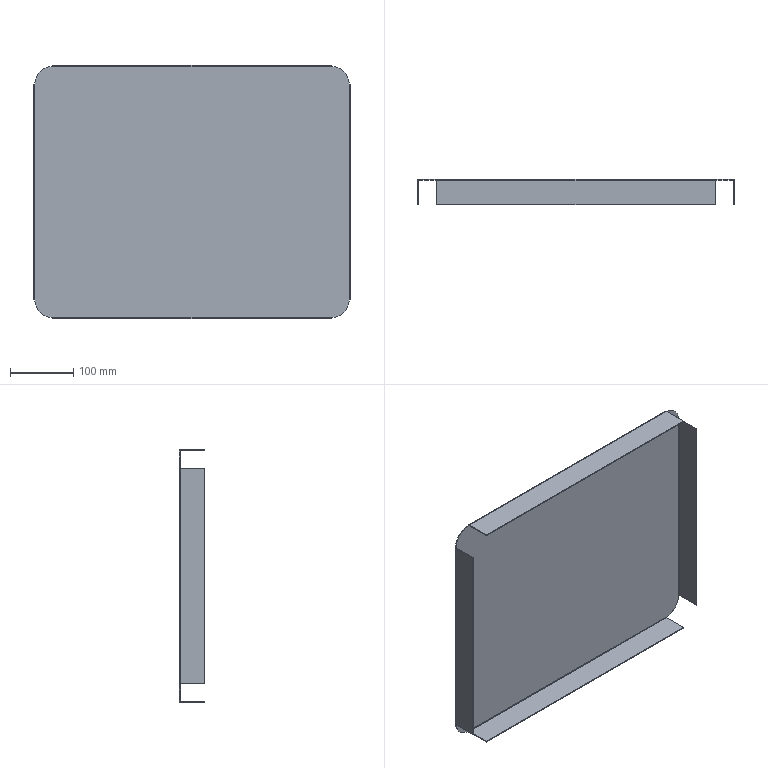Component | SolidWorks | dbj3-1_w11-1 | 1 solid | 42 faces | box 500 x 40 x 400 mm | volume 387129 mm3 | plane 30 | cylinder 12 | commonest cylinder face diameters 56 x4 4 x4 1 x4
STEP:
#1=COLOUR_RGB('',0.7922,0.8196,0.9333);
#2=FILL_AREA_STYLE_COLOUR('',#1);
#3=FILL_AREA_STYLE('',(#2));
#4=SURFACE_STYLE_FILL_AREA(#3);
#5=SURFACE_SIDE_STYLE('',(#4));
#6=SURFACE_STYLE_USAGE(.BOTH.,#5);
#7=PRESENTATION_STYLE_ASSIGNMENT((#6));
#8=CARTESIAN_POINT('',(-9.764,-29.498,8.661));
#9=VERTEX_POINT('',#8);
#10=CARTESIAN_POINT('',(-8.661,-29.498,9.764));
#11=VERTEX_POINT('',#10);
#12=CARTESIAN_POINT('',(-8.661,-29.498,8.661));
#13=DIRECTION('',(0.,1.,-0.));
#14=DIRECTION('',(1.,0.,0.));
#15=AXIS2_PLACEMENT_3D('',#12,#13,#14);
#16=CIRCLE('',#15,1.102);
#17=EDGE_CURVE('',#9,#11,#16,.T.);
#18=ORIENTED_EDGE('',*,*,#17,.F.);
#19=CARTESIAN_POINT('',(-9.764,-29.557,8.661));
#20=VERTEX_POINT('',#19);
#21=CARTESIAN_POINT('',(-9.764,-29.557,8.661));
#22=DIRECTION('',(0.,1.,-0.));
#23=VECTOR('',#22,39.37);
#24=LINE('',#21,#23);
#25=EDGE_CURVE('',#20,#9,#24,.T.);
#26=ORIENTED_EDGE('',*,*,#25,.F.);
#27=CARTESIAN_POINT('',(-8.661,-29.557,9.764));
#28=VERTEX_POINT('',#27);
#29=CARTESIAN_POINT('',(-8.661,-29.557,8.661));
#30=DIRECTION('',(0.,1.,-0.));
#31=DIRECTION('',(1.,0.,0.));
#32=AXIS2_PLACEMENT_3D('',#29,#30,#31);
#33=CIRCLE('',#32,1.102);
#34=EDGE_CURVE('',#20,#28,#33,.T.);
#35=ORIENTED_EDGE('',*,*,#34,.T.);
#36=CARTESIAN_POINT('',(-8.661,-29.557,9.764));
#37=DIRECTION('',(0.,1.,-0.));
#38=VECTOR('',#37,39.37);
#39=LINE('',#36,#38);
#40=EDGE_CURVE('',#28,#11,#39,.T.);
#41=ORIENTED_EDGE('',*,*,#40,.T.);
#42=EDGE_LOOP('',(#18,#26,#35,#41));
#43=FACE_OUTER_BOUND('',#42,.T.);
#44=CARTESIAN_POINT('',(-8.661,-29.557,8.661));
#45=DIRECTION('',(0.,1.,-0.));
#46=DIRECTION('',(1.,0.,0.));
#47=AXIS2_PLACEMENT_3D('',#44,#45,#46);
#48=CYLINDRICAL_SURFACE('',#47,1.102);
#49=ADVANCED_FACE('',(#43),#48,.T.);
#50=CARTESIAN_POINT('',(-8.661,-29.498,-5.827));
#51=VERTEX_POINT('',#50);
#52=CARTESIAN_POINT('',(-9.764,-29.498,-4.724));
#53=VERTEX_POINT('',#52);
#54=CARTESIAN_POINT('',(-8.661,-29.498,-4.724));
#55=DIRECTION('',(0.,1.,-0.));
#56=DIRECTION('',(1.,0.,0.));
#57=AXIS2_PLACEMENT_3D('',#54,#55,#56);
#58=CIRCLE('',#57,1.102);
#59=EDGE_CURVE('',#51,#53,#58,.T.);
#60=ORIENTED_EDGE('',*,*,#59,.F.);
#61=CARTESIAN_POINT('',(-8.661,-29.557,-5.827));
#62=VERTEX_POINT('',#61);
#63=CARTESIAN_POINT('',(-8.661,-29.557,-5.827));
#64=DIRECTION('',(0.,1.,-0.));
#65=VECTOR('',#64,39.37);
#66=LINE('',#63,#65);
#67=EDGE_CURVE('',#62,#51,#66,.T.);
#68=ORIENTED_EDGE('',*,*,#67,.F.);
#69=CARTESIAN_POINT('',(-9.764,-29.557,-4.724));
#70=VERTEX_POINT('',#69);
#71=CARTESIAN_POINT('',(-8.661,-29.557,-4.724));
#72=DIRECTION('',(0.,1.,-0.));
#73=DIRECTION('',(1.,0.,0.));
#74=AXIS2_PLACEMENT_3D('',#71,#72,#73);
#75=CIRCLE('',#74,1.102);
#76=EDGE_CURVE('',#62,#70,#75,.T.);
#77=ORIENTED_EDGE('',*,*,#76,.T.);
#78=CARTESIAN_POINT('',(-9.764,-29.557,-4.724));
#79=DIRECTION('',(0.,1.,-0.));
#80=VECTOR('',#79,39.37);
#81=LINE('',#78,#80);
#82=EDGE_CURVE('',#70,#53,#81,.T.);
#83=ORIENTED_EDGE('',*,*,#82,.T.);
#84=EDGE_LOOP('',(#60,#68,#77,#83));
#85=FACE_OUTER_BOUND('',#84,.T.);
#86=CARTESIAN_POINT('',(-8.661,-29.557,-4.724));
#87=DIRECTION('',(0.,1.,-0.));
#88=DIRECTION('',(1.,0.,0.));
#89=AXIS2_PLACEMENT_3D('',#86,#87,#88);
#90=CYLINDRICAL_SURFACE('',#89,1.102);
#91=ADVANCED_FACE('',(#85),#90,.T.);
#92=CARTESIAN_POINT('',(9.764,-29.498,-4.724));
#93=VERTEX_POINT('',#92);
#94=CARTESIAN_POINT('',(8.661,-29.498,-5.827));
#95=VERTEX_POINT('',#94);
#96=CARTESIAN_POINT('',(8.661,-29.498,-4.724));
#97=DIRECTION('',(0.,1.,-0.));
#98=DIRECTION('',(1.,0.,0.));
#99=AXIS2_PLACEMENT_3D('',#96,#97,#98);
#100=CIRCLE('',#99,1.102);
#101=EDGE_CURVE('',#93,#95,#100,.T.);
#102=ORIENTED_EDGE('',*,*,#101,.F.);
#103=CARTESIAN_POINT('',(9.764,-29.557,-4.724));
#104=VERTEX_POINT('',#103);
#105=CARTESIAN_POINT('',(9.764,-29.557,-4.724));
#106=DIRECTION('',(0.,1.,-0.));
#107=VECTOR('',#106,39.37);
#108=LINE('',#105,#107);
#109=EDGE_CURVE('',#104,#93,#108,.T.);
#110=ORIENTED_EDGE('',*,*,#109,.F.);
#111=CARTESIAN_POINT('',(8.661,-29.557,-5.827));
#112=VERTEX_POINT('',#111);
#113=CARTESIAN_POINT('',(8.661,-29.557,-4.724));
#114=DIRECTION('',(0.,1.,-0.));
#115=DIRECTION('',(1.,0.,0.));
#116=AXIS2_PLACEMENT_3D('',#113,#114,#115);
#117=CIRCLE('',#116,1.102);
#118=EDGE_CURVE('',#104,#112,#117,.T.);
#119=ORIENTED_EDGE('',*,*,#118,.T.);
#120=CARTESIAN_POINT('',(8.661,-29.557,-5.827));
#121=DIRECTION('',(0.,1.,-0.));
#122=VECTOR('',#121,39.37);
#123=LINE('',#120,#122);
#124=EDGE_CURVE('',#112,#95,#123,.T.);
#125=ORIENTED_EDGE('',*,*,#124,.T.);
#126=EDGE_LOOP('',(#102,#110,#119,#125));
#127=FACE_OUTER_BOUND('',#126,.T.);
#128=CARTESIAN_POINT('',(8.661,-29.557,-4.724));
#129=DIRECTION('',(0.,1.,-0.));
#130=DIRECTION('',(1.,0.,0.));
#131=AXIS2_PLACEMENT_3D('',#128,#129,#130);
#132=CYLINDRICAL_SURFACE('',#131,1.102);
#133=ADVANCED_FACE('',(#127),#132,.T.);
#134=CARTESIAN_POINT('',(8.661,-29.498,9.764));
#135=VERTEX_POINT('',#134);
#136=CARTESIAN_POINT('',(9.764,-29.498,8.661));
#137=VERTEX_POINT('',#136);
#138=CARTESIAN_POINT('',(8.661,-29.498,8.661));
#139=DIRECTION('',(0.,1.,-0.));
#140=DIRECTION('',(1.,0.,0.));
#141=AXIS2_PLACEMENT_3D('',#138,#139,#140);
#142=CIRCLE('',#141,1.102);
#143=EDGE_CURVE('',#135,#137,#142,.T.);
#144=ORIENTED_EDGE('',*,*,#143,.F.);
#145=CARTESIAN_POINT('',(8.661,-29.557,9.764));
#146=VERTEX_POINT('',#145);
#147=CARTESIAN_POINT('',(8.661,-29.557,9.764));
#148=DIRECTION('',(0.,1.,-0.));
#149=VECTOR('',#148,39.37);
#150=LINE('',#147,#149);
#151=EDGE_CURVE('',#146,#135,#150,.T.);
#152=ORIENTED_EDGE('',*,*,#151,.F.);
#153=CARTESIAN_POINT('',(9.764,-29.557,8.661));
#154=VERTEX_POINT('',#153);
#155=CARTESIAN_POINT('',(8.661,-29.557,8.661));
#156=DIRECTION('',(0.,1.,-0.));
#157=DIRECTION('',(1.,0.,0.));
#158=AXIS2_PLACEMENT_3D('',#155,#156,#157);
#159=CIRCLE('',#158,1.102);
#160=EDGE_CURVE('',#146,#154,#159,.T.);
#161=ORIENTED_EDGE('',*,*,#160,.T.);
#162=CARTESIAN_POINT('',(9.764,-29.557,8.661));
#163=DIRECTION('',(0.,1.,-0.));
#164=VECTOR('',#163,39.37);
#165=LINE('',#162,#164);
#166=EDGE_CURVE('',#154,#137,#165,.T.);
#167=ORIENTED_EDGE('',*,*,#166,.T.);
#168=EDGE_LOOP('',(#144,#152,#161,#167));
#169=FACE_OUTER_BOUND('',#168,.T.);
#170=CARTESIAN_POINT('',(8.661,-29.557,8.661));
#171=DIRECTION('',(0.,1.,-0.));
#172=DIRECTION('',(1.,0.,0.));
#173=AXIS2_PLACEMENT_3D('',#170,#171,#172);
#174=CYLINDRICAL_SURFACE('',#173,1.102);
#175=ADVANCED_FACE('',(#169),#174,.T.);
#176=ORIENTED_EDGE('',*,*,#34,.F.);
#177=CARTESIAN_POINT('',(-9.764,-29.557,8.661));
#178=DIRECTION('',(0.,0.,1.));
#179=VECTOR('',#178,39.37);
#180=LINE('',#177,#179);
#181=EDGE_CURVE('',#70,#20,#180,.T.);
#182=ORIENTED_EDGE('',*,*,#181,.F.);
#183=ORIENTED_EDGE('',*,*,#76,.F.);
#184=CARTESIAN_POINT('',(8.661,-29.557,-5.827));
#185=DIRECTION('',(-1.,0.,0.));
#186=VECTOR('',#185,39.37);
#187=LINE('',#184,#186);
#188=EDGE_CURVE('',#112,#62,#187,.T.);
#189=ORIENTED_EDGE('',*,*,#188,.F.);
#190=ORIENTED_EDGE('',*,*,#118,.F.);
#191=CARTESIAN_POINT('',(9.764,-29.557,8.661));
#192=DIRECTION('',(-0.,-0.,-1.));
#193=VECTOR('',#192,39.37);
#194=LINE('',#191,#193);
#195=EDGE_CURVE('',#154,#104,#194,.T.);
#196=ORIENTED_EDGE('',*,*,#195,.F.);
#197=ORIENTED_EDGE('',*,*,#160,.F.);
#198=CARTESIAN_POINT('',(8.661,-29.557,9.764));
#199=DIRECTION('',(1.,-0.,-0.));
#200=VECTOR('',#199,39.37);
#201=LINE('',#198,#200);
#202=EDGE_CURVE('',#28,#146,#201,.T.);
#203=ORIENTED_EDGE('',*,*,#202,.F.);
#204=EDGE_LOOP('',(#176,#182,#183,#189,#190,#196,#197,#203));
#205=FACE_OUTER_BOUND('',#204,.T.);
#206=CARTESIAN_POINT('',(-8.661,-29.557,8.661));
#207=DIRECTION('',(0.,1.,-0.));
#208=DIRECTION('',(1.,-0.,-0.));
#209=AXIS2_PLACEMENT_3D('',#206,#207,#208);
#210=PLANE('',#209);
#211=ADVANCED_FACE('',(#205),#210,.F.);
#212=ORIENTED_EDGE('',*,*,#17,.T.);
#213=CARTESIAN_POINT('',(8.661,-29.498,9.764));
#214=DIRECTION('',(1.,-0.,-0.));
#215=VECTOR('',#214,39.37);
#216=LINE('',#213,#215);
#217=EDGE_CURVE('',#11,#135,#216,.T.);
#218=ORIENTED_EDGE('',*,*,#217,.T.);
#219=ORIENTED_EDGE('',*,*,#143,.T.);
#220=CARTESIAN_POINT('',(9.764,-29.498,8.661));
#221=DIRECTION('',(-0.,-0.,-1.));
#222=VECTOR('',#221,39.37);
#223=LINE('',#220,#222);
#224=EDGE_CURVE('',#137,#93,#223,.T.);
#225=ORIENTED_EDGE('',*,*,#224,.T.);
#226=ORIENTED_EDGE('',*,*,#101,.T.);
#227=CARTESIAN_POINT('',(8.661,-29.498,-5.827));
#228=DIRECTION('',(-1.,0.,0.));
#229=VECTOR('',#228,39.37);
#230=LINE('',#227,#229);
#231=EDGE_CURVE('',#95,#51,#230,.T.);
#232=ORIENTED_EDGE('',*,*,#231,.T.);
#233=ORIENTED_EDGE('',*,*,#59,.T.);
#234=CARTESIAN_POINT('',(-9.764,-29.498,8.661));
#235=DIRECTION('',(0.,0.,1.));
#236=VECTOR('',#235,39.37);
#237=LINE('',#234,#236);
#238=EDGE_CURVE('',#53,#9,#237,.T.);
#239=ORIENTED_EDGE('',*,*,#238,.T.);
#240=EDGE_LOOP('',(#212,#218,#219,#225,#226,#232,#233,#239));
#241=FACE_OUTER_BOUND('',#240,.T.);
#242=CARTESIAN_POINT('',(-8.661,-29.498,8.661));
#243=DIRECTION('',(0.,1.,-0.));
#244=DIRECTION('',(1.,-0.,-0.));
#245=AXIS2_PLACEMENT_3D('',#242,#243,#244);
#246=PLANE('',#245);
#247=ADVANCED_FACE('',(#241),#246,.T.);
#248=CARTESIAN_POINT('',(-8.661,-29.577,-5.846));
#249=VERTEX_POINT('',#248);
#250=CARTESIAN_POINT('',(-8.661,-29.577,-5.906));
#251=VERTEX_POINT('',#250);
#252=CARTESIAN_POINT('',(-8.661,-29.577,-5.906));
#253=DIRECTION('',(-0.,0.,-1.));
#254=VECTOR('',#253,39.37);
#255=LINE('',#252,#254);
#256=EDGE_CURVE('',#249,#251,#255,.T.);
#257=ORIENTED_EDGE('',*,*,#256,.F.);
#258=CARTESIAN_POINT('',(-8.661,-29.577,-5.827));
#259=DIRECTION('',(-1.,0.,0.));
#260=DIRECTION('',(0.,-1.,0.));
#261=AXIS2_PLACEMENT_3D('',#258,#259,#260);
#262=CIRCLE('',#261,0.01969);
#263=EDGE_CURVE('',#62,#249,#262,.T.);
#264=ORIENTED_EDGE('',*,*,#263,.F.);
#265=ORIENTED_EDGE('',*,*,#67,.T.);
#266=CARTESIAN_POINT('',(-8.661,-29.577,-5.827));
#267=DIRECTION('',(-1.,0.,0.));
#268=DIRECTION('',(0.,-1.,0.));
#269=AXIS2_PLACEMENT_3D('',#266,#267,#268);
#270=CIRCLE('',#269,0.07874);
#271=EDGE_CURVE('',#51,#251,#270,.T.);
#272=ORIENTED_EDGE('',*,*,#271,.T.);
#273=EDGE_LOOP('',(#257,#264,#265,#272));
#274=FACE_OUTER_BOUND('',#273,.T.);
#275=CARTESIAN_POINT('',(-8.661,-29.577,-5.827));
#276=DIRECTION('',(-1.,0.,0.));
#277=DIRECTION('',(0.,1.,-0.));
#278=AXIS2_PLACEMENT_3D('',#275,#276,#277);
#279=PLANE('',#278);
#280=ADVANCED_FACE('',(#274),#279,.T.);
#281=CARTESIAN_POINT('',(8.661,-29.577,-5.846));
#282=VERTEX_POINT('',#281);
#283=CARTESIAN_POINT('',(8.661,-29.577,-5.827));
#284=DIRECTION('',(1.,-0.,-0.));
#285=DIRECTION('',(0.,-1.,0.));
#286=AXIS2_PLACEMENT_3D('',#283,#284,#285);
#287=CIRCLE('',#286,0.01969);
#288=EDGE_CURVE('',#282,#112,#287,.T.);
#289=ORIENTED_EDGE('',*,*,#288,.F.);
#290=CARTESIAN_POINT('',(8.661,-29.577,-5.906));
#291=VERTEX_POINT('',#290);
#292=CARTESIAN_POINT('',(8.661,-29.577,-5.846));
#293=DIRECTION('',(-0.,0.,-1.));
#294=VECTOR('',#293,39.37);
#295=LINE('',#292,#294);
#296=EDGE_CURVE('',#282,#291,#295,.T.);
#297=ORIENTED_EDGE('',*,*,#296,.T.);
#298=CARTESIAN_POINT('',(8.661,-29.577,-5.827));
#299=DIRECTION('',(1.,-0.,-0.));
#300=DIRECTION('',(0.,-1.,0.));
#301=AXIS2_PLACEMENT_3D('',#298,#299,#300);
#302=CIRCLE('',#301,0.07874);
#303=EDGE_CURVE('',#291,#95,#302,.T.);
#304=ORIENTED_EDGE('',*,*,#303,.T.);
#305=ORIENTED_EDGE('',*,*,#124,.F.);
#306=EDGE_LOOP('',(#289,#297,#304,#305));
#307=FACE_OUTER_BOUND('',#306,.T.);
#308=CARTESIAN_POINT('',(8.661,-29.577,-5.827));
#309=DIRECTION('',(-1.,0.,0.));
#310=DIRECTION('',(0.,1.,-0.));
#311=AXIS2_PLACEMENT_3D('',#308,#309,#310);
#312=PLANE('',#311);
#313=ADVANCED_FACE('',(#307),#312,.F.);
#314=ORIENTED_EDGE('',*,*,#231,.F.);
#315=ORIENTED_EDGE('',*,*,#303,.F.);
#316=CARTESIAN_POINT('',(-8.661,-29.577,-5.906));
#317=DIRECTION('',(-1.,0.,0.));
#318=VECTOR('',#317,39.37);
#319=LINE('',#316,#318);
#320=EDGE_CURVE('',#291,#251,#319,.T.);
#321=ORIENTED_EDGE('',*,*,#320,.T.);
#322=ORIENTED_EDGE('',*,*,#271,.F.);
#323=EDGE_LOOP('',(#314,#315,#321,#322));
#324=FACE_OUTER_BOUND('',#323,.T.);
#325=CARTESIAN_POINT('',(8.661,-29.577,-5.827));
#326=DIRECTION('',(1.,-0.,-0.));
#327=DIRECTION('',(0.,0.,-1.));
#328=AXIS2_PLACEMENT_3D('',#325,#326,#327);
#329=CYLINDRICAL_SURFACE('',#328,0.07874);
#330=ADVANCED_FACE('',(#324),#329,.T.);
#331=ORIENTED_EDGE('',*,*,#188,.T.);
#332=ORIENTED_EDGE('',*,*,#263,.T.);
#333=CARTESIAN_POINT('',(-8.661,-29.577,-5.846));
#334=DIRECTION('',(1.,-0.,-0.));
#335=VECTOR('',#334,39.37);
#336=LINE('',#333,#335);
#337=EDGE_CURVE('',#249,#282,#336,.T.);
#338=ORIENTED_EDGE('',*,*,#337,.T.);
#339=ORIENTED_EDGE('',*,*,#288,.T.);
#340=EDGE_LOOP('',(#331,#332,#338,#339));
#341=FACE_OUTER_BOUND('',#340,.T.);
#342=CARTESIAN_POINT('',(8.661,-29.577,-5.827));
#343=DIRECTION('',(1.,-0.,-0.));
#344=DIRECTION('',(0.,0.,-1.));
#345=AXIS2_PLACEMENT_3D('',#342,#343,#344);
#346=CYLINDRICAL_SURFACE('',#345,0.01969);
#347=ADVANCED_FACE('',(#341),#346,.F.);
#348=ORIENTED_EDGE('',*,*,#296,.F.);
#349=CARTESIAN_POINT('',(8.661,-31.073,-5.846));
#350=VERTEX_POINT('',#349);
#351=CARTESIAN_POINT('',(8.661,-31.073,-5.846));
#352=DIRECTION('',(-0.,-1.,-0.));
#353=VECTOR('',#352,39.37);
#354=LINE('',#351,#353);
#355=EDGE_CURVE('',#282,#350,#354,.T.);
#356=ORIENTED_EDGE('',*,*,#355,.T.);
#357=CARTESIAN_POINT('',(8.661,-31.073,-5.906));
#358=VERTEX_POINT('',#357);
#359=CARTESIAN_POINT('',(8.661,-31.073,-5.906));
#360=DIRECTION('',(0.,0.,1.));
#361=VECTOR('',#360,39.37);
#362=LINE('',#359,#361);
#363=EDGE_CURVE('',#358,#350,#362,.T.);
#364=ORIENTED_EDGE('',*,*,#363,.F.);
#365=CARTESIAN_POINT('',(8.661,-29.498,-5.906));
#366=DIRECTION('',(-0.,-1.,-0.));
#367=VECTOR('',#366,39.37);
#368=LINE('',#365,#367);
#369=EDGE_CURVE('',#291,#358,#368,.T.);
#370=ORIENTED_EDGE('',*,*,#369,.F.);
#371=EDGE_LOOP('',(#348,#356,#364,#370));
#372=FACE_OUTER_BOUND('',#371,.T.);
#373=CARTESIAN_POINT('',(8.661,-31.073,-5.906));
#374=DIRECTION('',(-1.,0.,0.));
#375=DIRECTION('',(0.,0.,1.));
#376=AXIS2_PLACEMENT_3D('',#373,#374,#375);
#377=PLANE('',#376);
#378=ADVANCED_FACE('',(#372),#377,.F.);
#379=ORIENTED_EDGE('',*,*,#256,.T.);
#380=CARTESIAN_POINT('',(-8.661,-31.073,-5.906));
#381=VERTEX_POINT('',#380);
#382=CARTESIAN_POINT('',(-8.661,-29.498,-5.906));
#383=DIRECTION('',(0.,1.,0.));
#384=VECTOR('',#383,39.37);
#385=LINE('',#382,#384);
#386=EDGE_CURVE('',#381,#251,#385,.T.);
#387=ORIENTED_EDGE('',*,*,#386,.F.);
#388=CARTESIAN_POINT('',(-8.661,-31.073,-5.846));
#389=VERTEX_POINT('',#388);
#390=CARTESIAN_POINT('',(-8.661,-31.073,-5.906));
#391=DIRECTION('',(0.,0.,1.));
#392=VECTOR('',#391,39.37);
#393=LINE('',#390,#392);
#394=EDGE_CURVE('',#381,#389,#393,.T.);
#395=ORIENTED_EDGE('',*,*,#394,.T.);
#396=CARTESIAN_POINT('',(-8.661,-29.557,-5.846));
#397=DIRECTION('',(0.,1.,0.));
#398=VECTOR('',#397,39.37);
#399=LINE('',#396,#398);
#400=EDGE_CURVE('',#389,#249,#399,.T.);
#401=ORIENTED_EDGE('',*,*,#400,.T.);
#402=EDGE_LOOP('',(#379,#387,#395,#401));
#403=FACE_OUTER_BOUND('',#402,.T.);
#404=CARTESIAN_POINT('',(-8.661,-29.557,-5.906));
#405=DIRECTION('',(1.,-0.,-0.));
#406=DIRECTION('',(-0.,-0.,-1.));
#407=AXIS2_PLACEMENT_3D('',#404,#405,#406);
#408=PLANE('',#407);
#409=ADVANCED_FACE('',(#403),#408,.F.);
#410=ORIENTED_EDGE('',*,*,#320,.F.);
#411=ORIENTED_EDGE('',*,*,#369,.T.);
#412=CARTESIAN_POINT('',(0.,-31.073,-5.906));
#413=DIRECTION('',(-1.,0.,0.));
#414=VECTOR('',#413,39.37);
#415=LINE('',#412,#414);
#416=EDGE_CURVE('',#358,#381,#415,.T.);
#417=ORIENTED_EDGE('',*,*,#416,.T.);
#418=ORIENTED_EDGE('',*,*,#386,.T.);
#419=EDGE_LOOP('',(#410,#411,#417,#418));
#420=FACE_OUTER_BOUND('',#419,.T.);
#421=CARTESIAN_POINT('',(0.,-29.498,-5.906));
#422=DIRECTION('',(0.,-0.,1.));
#423=DIRECTION('',(-0.,-1.,-0.));
#424=AXIS2_PLACEMENT_3D('',#421,#422,#423);
#425=PLANE('',#424);
#426=ADVANCED_FACE('',(#420),#425,.F.);
#427=ORIENTED_EDGE('',*,*,#355,.F.);
#428=ORIENTED_EDGE('',*,*,#337,.F.);
#429=ORIENTED_EDGE('',*,*,#400,.F.);
#430=CARTESIAN_POINT('',(-8.661,-31.073,-5.846));
#431=DIRECTION('',(-1.,0.,0.));
#432=VECTOR('',#431,39.37);
#433=LINE('',#430,#432);
#434=EDGE_CURVE('',#350,#389,#433,.T.);
#435=ORIENTED_EDGE('',*,*,#434,.F.);
#436=EDGE_LOOP('',(#427,#428,#429,#435));
#437=FACE_OUTER_BOUND('',#436,.T.);
#438=CARTESIAN_POINT('',(0.,-29.498,-5.846));
#439=DIRECTION('',(0.,-0.,1.));
#440=DIRECTION('',(-0.,-1.,-0.));
#441=AXIS2_PLACEMENT_3D('',#438,#439,#440);
#442=PLANE('',#441);
#443=ADVANCED_FACE('',(#437),#442,.T.);
#444=ORIENTED_EDGE('',*,*,#434,.T.);
#445=ORIENTED_EDGE('',*,*,#394,.F.);
#446=ORIENTED_EDGE('',*,*,#416,.F.);
#447=ORIENTED_EDGE('',*,*,#363,.T.);
#448=EDGE_LOOP('',(#444,#445,#446,#447));
#449=FACE_OUTER_BOUND('',#448,.T.);
#450=CARTESIAN_POINT('',(-8.661,-31.073,-5.906));
#451=DIRECTION('',(0.,1.,-0.));
#452=DIRECTION('',(0.,0.,1.));
#453=AXIS2_PLACEMENT_3D('',#450,#451,#452);
#454=PLANE('',#453);
#455=ADVANCED_FACE('',(#449),#454,.F.);
#456=CARTESIAN_POINT('',(-9.783,-29.577,8.661));
#457=VERTEX_POINT('',#456);
#458=CARTESIAN_POINT('',(-9.843,-29.577,8.661));
#459=VERTEX_POINT('',#458);
#460=CARTESIAN_POINT('',(-9.843,-29.577,8.661));
#461=DIRECTION('',(-1.,0.,-0.));
#462=VECTOR('',#461,39.37);
#463=LINE('',#460,#462);
#464=EDGE_CURVE('',#457,#459,#463,.T.);
#465=ORIENTED_EDGE('',*,*,#464,.F.);
#466=CARTESIAN_POINT('',(-9.764,-29.577,8.661));
#467=DIRECTION('',(0.,0.,1.));
#468=DIRECTION('',(0.,1.,0.));
#469=AXIS2_PLACEMENT_3D('',#466,#467,#468);
#470=CIRCLE('',#469,0.01969);
#471=EDGE_CURVE('',#20,#457,#470,.T.);
#472=ORIENTED_EDGE('',*,*,#471,.F.);
#473=ORIENTED_EDGE('',*,*,#25,.T.);
#474=CARTESIAN_POINT('',(-9.764,-29.577,8.661));
#475=DIRECTION('',(0.,0.,1.));
#476=DIRECTION('',(0.,1.,0.));
#477=AXIS2_PLACEMENT_3D('',#474,#475,#476);
#478=CIRCLE('',#477,0.07874);
#479=EDGE_CURVE('',#9,#459,#478,.T.);
#480=ORIENTED_EDGE('',*,*,#479,.T.);
#481=EDGE_LOOP('',(#465,#472,#473,#480));
#482=FACE_OUTER_BOUND('',#481,.T.);
#483=CARTESIAN_POINT('',(-9.764,-29.577,8.661));
#484=DIRECTION('',(0.,0.,1.));
#485=DIRECTION('',(-0.,-1.,0.));
#486=AXIS2_PLACEMENT_3D('',#483,#484,#485);
#487=PLANE('',#486);
#488=ADVANCED_FACE('',(#482),#487,.T.);
#489=CARTESIAN_POINT('',(-9.783,-29.577,-4.724));
#490=VERTEX_POINT('',#489);
#491=CARTESIAN_POINT('',(-9.764,-29.577,-4.724));
#492=DIRECTION('',(-0.,-0.,-1.));
#493=DIRECTION('',(0.,1.,0.));
#494=AXIS2_PLACEMENT_3D('',#491,#492,#493);
#495=CIRCLE('',#494,0.01969);
#496=EDGE_CURVE('',#490,#70,#495,.T.);
#497=ORIENTED_EDGE('',*,*,#496,.F.);
#498=CARTESIAN_POINT('',(-9.843,-29.577,-4.724));
#499=VERTEX_POINT('',#498);
#500=CARTESIAN_POINT('',(-9.783,-29.577,-4.724));
#501=DIRECTION('',(-1.,0.,-0.));
#502=VECTOR('',#501,39.37);
#503=LINE('',#500,#502);
#504=EDGE_CURVE('',#490,#499,#503,.T.);
#505=ORIENTED_EDGE('',*,*,#504,.T.);
#506=CARTESIAN_POINT('',(-9.764,-29.577,-4.724));
#507=DIRECTION('',(-0.,-0.,-1.));
#508=DIRECTION('',(0.,1.,-0.));
#509=AXIS2_PLACEMENT_3D('',#506,#507,#508);
#510=CIRCLE('',#509,0.07874);
#511=EDGE_CURVE('',#499,#53,#510,.T.);
#512=ORIENTED_EDGE('',*,*,#511,.T.);
#513=ORIENTED_EDGE('',*,*,#82,.F.);
#514=EDGE_LOOP('',(#497,#505,#512,#513));
#515=FACE_OUTER_BOUND('',#514,.T.);
#516=CARTESIAN_POINT('',(-9.764,-29.577,-4.724));
#517=DIRECTION('',(0.,0.,1.));
#518=DIRECTION('',(-0.,-1.,0.));
#519=AXIS2_PLACEMENT_3D('',#516,#517,#518);
#520=PLANE('',#519);
#521=ADVANCED_FACE('',(#515),#520,.F.);
#522=ORIENTED_EDGE('',*,*,#238,.F.);
#523=ORIENTED_EDGE('',*,*,#511,.F.);
#524=CARTESIAN_POINT('',(-9.843,-29.577,8.661));
#525=DIRECTION('',(0.,0.,1.));
#526=VECTOR('',#525,39.37);
#527=LINE('',#524,#526);
#528=EDGE_CURVE('',#499,#459,#527,.T.);
#529=ORIENTED_EDGE('',*,*,#528,.T.);
#530=ORIENTED_EDGE('',*,*,#479,.F.);
#531=EDGE_LOOP('',(#522,#523,#529,#530));
#532=FACE_OUTER_BOUND('',#531,.T.);
#533=CARTESIAN_POINT('',(-9.764,-29.577,-4.724));
#534=DIRECTION('',(-0.,-0.,-1.));
#535=DIRECTION('',(-1.,0.,0.));
#536=AXIS2_PLACEMENT_3D('',#533,#534,#535);
#537=CYLINDRICAL_SURFACE('',#536,0.07874);
#538=ADVANCED_FACE('',(#532),#537,.T.);
#539=ORIENTED_EDGE('',*,*,#181,.T.);
#540=ORIENTED_EDGE('',*,*,#471,.T.);
#541=CARTESIAN_POINT('',(-9.783,-29.577,8.661));
#542=DIRECTION('',(-0.,-0.,-1.));
#543=VECTOR('',#542,39.37);
#544=LINE('',#541,#543);
#545=EDGE_CURVE('',#457,#490,#544,.T.);
#546=ORIENTED_EDGE('',*,*,#545,.T.);
#547=ORIENTED_EDGE('',*,*,#496,.T.);
#548=EDGE_LOOP('',(#539,#540,#546,#547));
#549=FACE_OUTER_BOUND('',#548,.T.);
#550=CARTESIAN_POINT('',(-9.764,-29.577,-4.724));
#551=DIRECTION('',(-0.,-0.,-1.));
#552=DIRECTION('',(-1.,0.,0.));
#553=AXIS2_PLACEMENT_3D('',#550,#551,#552);
#554=CYLINDRICAL_SURFACE('',#553,0.01969);
#555=ADVANCED_FACE('',(#549),#554,.F.);
#556=ORIENTED_EDGE('',*,*,#504,.F.);
#557=CARTESIAN_POINT('',(-9.783,-31.073,-4.724));
#558=VERTEX_POINT('',#557);
#559=CARTESIAN_POINT('',(-9.783,-31.073,-4.724));
#560=DIRECTION('',(-0.,-1.,0.));
#561=VECTOR('',#560,39.37);
#562=LINE('',#559,#561);
#563=EDGE_CURVE('',#490,#558,#562,.T.);
#564=ORIENTED_EDGE('',*,*,#563,.T.);
#565=CARTESIAN_POINT('',(-9.843,-31.073,-4.724));
#566=VERTEX_POINT('',#565);
#567=CARTESIAN_POINT('',(-9.843,-31.073,-4.724));
#568=DIRECTION('',(1.,-0.,0.));
#569=VECTOR('',#568,39.37);
#570=LINE('',#567,#569);
#571=EDGE_CURVE('',#566,#558,#570,.T.);
#572=ORIENTED_EDGE('',*,*,#571,.F.);
#573=CARTESIAN_POINT('',(-9.843,-29.498,-4.724));
#574=DIRECTION('',(-0.,-1.,0.));
#575=VECTOR('',#574,39.37);
#576=LINE('',#573,#575);
#577=EDGE_CURVE('',#499,#566,#576,.T.);
#578=ORIENTED_EDGE('',*,*,#577,.F.);
#579=EDGE_LOOP('',(#556,#564,#572,#578));
#580=FACE_OUTER_BOUND('',#579,.T.);
#581=CARTESIAN_POINT('',(-9.843,-31.073,-4.724));
#582=DIRECTION('',(0.,0.,1.));
#583=DIRECTION('',(-0.,-1.,0.));
#584=AXIS2_PLACEMENT_3D('',#581,#582,#583);
#585=PLANE('',#584);
#586=ADVANCED_FACE('',(#580),#585,.F.);
#587=ORIENTED_EDGE('',*,*,#464,.T.);
#588=CARTESIAN_POINT('',(-9.843,-31.073,8.661));
#589=VERTEX_POINT('',#588);
#590=CARTESIAN_POINT('',(-9.843,-29.498,8.661));
#591=DIRECTION('',(0.,1.,-0.));
#592=VECTOR('',#591,39.37);
#593=LINE('',#590,#592);
#594=EDGE_CURVE('',#589,#459,#593,.T.);
#595=ORIENTED_EDGE('',*,*,#594,.F.);
#596=CARTESIAN_POINT('',(-9.783,-31.073,8.661));
#597=VERTEX_POINT('',#596);
#598=CARTESIAN_POINT('',(-9.843,-31.073,8.661));
#599=DIRECTION('',(1.,-0.,0.));
#600=VECTOR('',#599,39.37);
#601=LINE('',#598,#600);
#602=EDGE_CURVE('',#589,#597,#601,.T.);
#603=ORIENTED_EDGE('',*,*,#602,.T.);
#604=CARTESIAN_POINT('',(-9.783,-29.557,8.661));
#605=DIRECTION('',(0.,1.,-0.));
#606=VECTOR('',#605,39.37);
#607=LINE('',#604,#606);
#608=EDGE_CURVE('',#597,#457,#607,.T.);
#609=ORIENTED_EDGE('',*,*,#608,.T.);
#610=EDGE_LOOP('',(#587,#595,#603,#609));
#611=FACE_OUTER_BOUND('',#610,.T.);
#612=CARTESIAN_POINT('',(-9.843,-29.557,8.661));
#613=DIRECTION('',(-0.,-0.,-1.));
#614=DIRECTION('',(0.,1.,-0.));
#615=AXIS2_PLACEMENT_3D('',#612,#613,#614);
#616=PLANE('',#615);
#617=ADVANCED_FACE('',(#611),#616,.F.);
#618=ORIENTED_EDGE('',*,*,#528,.F.);
#619=ORIENTED_EDGE('',*,*,#577,.T.);
#620=CARTESIAN_POINT('',(-9.843,-31.073,1.969));
#621=DIRECTION('',(0.,0.,1.));
#622=VECTOR('',#621,39.37);
#623=LINE('',#620,#622);
#624=EDGE_CURVE('',#566,#589,#623,.T.);
#625=ORIENTED_EDGE('',*,*,#624,.T.);
#626=ORIENTED_EDGE('',*,*,#594,.T.);
#627=EDGE_LOOP('',(#618,#619,#625,#626));
#628=FACE_OUTER_BOUND('',#627,.T.);
#629=CARTESIAN_POINT('',(-9.843,-29.498,1.969));
#630=DIRECTION('',(1.,-0.,0.));
#631=DIRECTION('',(-0.,-1.,0.));
#632=AXIS2_PLACEMENT_3D('',#629,#630,#631);
#633=PLANE('',#632);
#634=ADVANCED_FACE('',(#628),#633,.F.);
#635=ORIENTED_EDGE('',*,*,#563,.F.);
#636=ORIENTED_EDGE('',*,*,#545,.F.);
#637=ORIENTED_EDGE('',*,*,#608,.F.);
#638=CARTESIAN_POINT('',(-9.783,-31.073,8.661));
#639=DIRECTION('',(0.,0.,1.));
#640=VECTOR('',#639,39.37);
#641=LINE('',#638,#640);
#642=EDGE_CURVE('',#558,#597,#641,.T.);
#643=ORIENTED_EDGE('',*,*,#642,.F.);
#644=EDGE_LOOP('',(#635,#636,#637,#643));
#645=FACE_OUTER_BOUND('',#644,.T.);
#646=CARTESIAN_POINT('',(-9.783,-29.498,1.969));
#647=DIRECTION('',(1.,-0.,0.));
#648=DIRECTION('',(-0.,-1.,0.));
#649=AXIS2_PLACEMENT_3D('',#646,#647,#648);
#650=PLANE('',#649);
#651=ADVANCED_FACE('',(#645),#650,.T.);
#652=ORIENTED_EDGE('',*,*,#642,.T.);
#653=ORIENTED_EDGE('',*,*,#602,.F.);
#654=ORIENTED_EDGE('',*,*,#624,.F.);
#655=ORIENTED_EDGE('',*,*,#571,.T.);
#656=EDGE_LOOP('',(#652,#653,#654,#655));
#657=FACE_OUTER_BOUND('',#656,.T.);
#658=CARTESIAN_POINT('',(-9.843,-31.073,8.661));
#659=DIRECTION('',(0.,1.,-0.));
#660=DIRECTION('',(1.,-0.,0.));
#661=AXIS2_PLACEMENT_3D('',#658,#659,#660);
#662=PLANE('',#661);
#663=ADVANCED_FACE('',(#657),#662,.F.);
#664=CARTESIAN_POINT('',(9.783,-29.577,-4.724));
#665=VERTEX_POINT('',#664);
#666=CARTESIAN_POINT('',(9.843,-29.577,-4.724));
#667=VERTEX_POINT('',#666);
#668=CARTESIAN_POINT('',(9.843,-29.577,-4.724));
#669=DIRECTION('',(1.,0.,-0.));
#670=VECTOR('',#669,39.37);
#671=LINE('',#668,#670);
#672=EDGE_CURVE('',#665,#667,#671,.T.);
#673=ORIENTED_EDGE('',*,*,#672,.F.);
#674=CARTESIAN_POINT('',(9.764,-29.577,-4.724));
#675=DIRECTION('',(-0.,-0.,-1.));
#676=DIRECTION('',(0.,-1.,0.));
#677=AXIS2_PLACEMENT_3D('',#674,#675,#676);
#678=CIRCLE('',#677,0.01969);
#679=EDGE_CURVE('',#104,#665,#678,.T.);
#680=ORIENTED_EDGE('',*,*,#679,.F.);
#681=ORIENTED_EDGE('',*,*,#109,.T.);
#682=CARTESIAN_POINT('',(9.764,-29.577,-4.724));
#683=DIRECTION('',(-0.,-0.,-1.));
#684=DIRECTION('',(0.,-1.,0.));
#685=AXIS2_PLACEMENT_3D('',#682,#683,#684);
#686=CIRCLE('',#685,0.07874);
#687=EDGE_CURVE('',#93,#667,#686,.T.);
#688=ORIENTED_EDGE('',*,*,#687,.T.);
#689=EDGE_LOOP('',(#673,#680,#681,#688));
#690=FACE_OUTER_BOUND('',#689,.T.);
#691=CARTESIAN_POINT('',(9.764,-29.577,-4.724));
#692=DIRECTION('',(-0.,-0.,-1.));
#693=DIRECTION('',(0.,1.,-0.));
#694=AXIS2_PLACEMENT_3D('',#691,#692,#693);
#695=PLANE('',#694);
#696=ADVANCED_FACE('',(#690),#695,.T.);
#697=CARTESIAN_POINT('',(9.783,-29.577,8.661));
#698=VERTEX_POINT('',#697);
#699=CARTESIAN_POINT('',(9.764,-29.577,8.661));
#700=DIRECTION('',(0.,0.,1.));
#701=DIRECTION('',(0.,-1.,0.));
#702=AXIS2_PLACEMENT_3D('',#699,#700,#701);
#703=CIRCLE('',#702,0.01969);
#704=EDGE_CURVE('',#698,#154,#703,.T.);
#705=ORIENTED_EDGE('',*,*,#704,.F.);
#706=CARTESIAN_POINT('',(9.843,-29.577,8.661));
#707=VERTEX_POINT('',#706);
#708=CARTESIAN_POINT('',(9.783,-29.577,8.661));
#709=DIRECTION('',(1.,0.,-0.));
#710=VECTOR('',#709,39.37);
#711=LINE('',#708,#710);
#712=EDGE_CURVE('',#698,#707,#711,.T.);
#713=ORIENTED_EDGE('',*,*,#712,.T.);
#714=CARTESIAN_POINT('',(9.764,-29.577,8.661));
#715=DIRECTION('',(0.,0.,1.));
#716=DIRECTION('',(0.,-1.,0.));
#717=AXIS2_PLACEMENT_3D('',#714,#715,#716);
#718=CIRCLE('',#717,0.07874);
#719=EDGE_CURVE('',#707,#137,#718,.T.);
#720=ORIENTED_EDGE('',*,*,#719,.T.);
#721=ORIENTED_EDGE('',*,*,#166,.F.);
#722=EDGE_LOOP('',(#705,#713,#720,#721));
#723=FACE_OUTER_BOUND('',#722,.T.);
#724=CARTESIAN_POINT('',(9.764,-29.577,8.661));
#725=DIRECTION('',(-0.,-0.,-1.));
#726=DIRECTION('',(0.,1.,-0.));
#727=AXIS2_PLACEMENT_3D('',#724,#725,#726);
#728=PLANE('',#727);
#729=ADVANCED_FACE('',(#723),#728,.F.);
#730=ORIENTED_EDGE('',*,*,#224,.F.);
#731=ORIENTED_EDGE('',*,*,#719,.F.);
#732=CARTESIAN_POINT('',(9.843,-29.577,-4.724));
#733=DIRECTION('',(-0.,-0.,-1.));
#734=VECTOR('',#733,39.37);
#735=LINE('',#732,#734);
#736=EDGE_CURVE('',#707,#667,#735,.T.);
#737=ORIENTED_EDGE('',*,*,#736,.T.);
#738=ORIENTED_EDGE('',*,*,#687,.F.);
#739=EDGE_LOOP('',(#730,#731,#737,#738));
#740=FACE_OUTER_BOUND('',#739,.T.);
#741=CARTESIAN_POINT('',(9.764,-29.577,8.661));
#742=DIRECTION('',(0.,0.,1.));
#743=DIRECTION('',(1.,0.,0.));
#744=AXIS2_PLACEMENT_3D('',#741,#742,#743);
#745=CYLINDRICAL_SURFACE('',#744,0.07874);
#746=ADVANCED_FACE('',(#740),#745,.T.);
#747=ORIENTED_EDGE('',*,*,#195,.T.);
#748=ORIENTED_EDGE('',*,*,#679,.T.);
#749=CARTESIAN_POINT('',(9.783,-29.577,-4.724));
#750=DIRECTION('',(0.,0.,1.));
#751=VECTOR('',#750,39.37);
#752=LINE('',#749,#751);
#753=EDGE_CURVE('',#665,#698,#752,.T.);
#754=ORIENTED_EDGE('',*,*,#753,.T.);
#755=ORIENTED_EDGE('',*,*,#704,.T.);
#756=EDGE_LOOP('',(#747,#748,#754,#755));
#757=FACE_OUTER_BOUND('',#756,.T.);
#758=CARTESIAN_POINT('',(9.764,-29.577,8.661));
#759=DIRECTION('',(0.,0.,1.));
#760=DIRECTION('',(1.,0.,0.));
#761=AXIS2_PLACEMENT_3D('',#758,#759,#760);
#762=CYLINDRICAL_SURFACE('',#761,0.01969);
#763=ADVANCED_FACE('',(#757),#762,.F.);
#764=ORIENTED_EDGE('',*,*,#712,.F.);
#765=CARTESIAN_POINT('',(9.783,-31.073,8.661));
#766=VERTEX_POINT('',#765);
#767=CARTESIAN_POINT('',(9.783,-31.073,8.661));
#768=DIRECTION('',(0.,-1.,0.));
#769=VECTOR('',#768,39.37);
#770=LINE('',#767,#769);
#771=EDGE_CURVE('',#698,#766,#770,.T.);
#772=ORIENTED_EDGE('',*,*,#771,.T.);
#773=CARTESIAN_POINT('',(9.843,-31.073,8.661));
#774=VERTEX_POINT('',#773);
#775=CARTESIAN_POINT('',(9.843,-31.073,8.661));
#776=DIRECTION('',(-1.,-0.,0.));
#777=VECTOR('',#776,39.37);
#778=LINE('',#775,#777);
#779=EDGE_CURVE('',#774,#766,#778,.T.);
#780=ORIENTED_EDGE('',*,*,#779,.F.);
#781=CARTESIAN_POINT('',(9.843,-29.498,8.661));
#782=DIRECTION('',(0.,-1.,0.));
#783=VECTOR('',#782,39.37);
#784=LINE('',#781,#783);
#785=EDGE_CURVE('',#707,#774,#784,.T.);
#786=ORIENTED_EDGE('',*,*,#785,.F.);
#787=EDGE_LOOP('',(#764,#772,#780,#786));
#788=FACE_OUTER_BOUND('',#787,.T.);
#789=CARTESIAN_POINT('',(9.843,-31.073,8.661));
#790=DIRECTION('',(-0.,-0.,-1.));
#791=DIRECTION('',(0.,1.,-0.));
#792=AXIS2_PLACEMENT_3D('',#789,#790,#791);
#793=PLANE('',#792);
#794=ADVANCED_FACE('',(#788),#793,.F.);
#795=ORIENTED_EDGE('',*,*,#672,.T.);
#796=CARTESIAN_POINT('',(9.843,-31.073,-4.724));
#797=VERTEX_POINT('',#796);
#798=CARTESIAN_POINT('',(9.843,-29.498,-4.724));
#799=DIRECTION('',(-0.,1.,-0.));
#800=VECTOR('',#799,39.37);
#801=LINE('',#798,#800);
#802=EDGE_CURVE('',#797,#667,#801,.T.);
#803=ORIENTED_EDGE('',*,*,#802,.F.);
#804=CARTESIAN_POINT('',(9.783,-31.073,-4.724));
#805=VERTEX_POINT('',#804);
#806=CARTESIAN_POINT('',(9.843,-31.073,-4.724));
#807=DIRECTION('',(-1.,-0.,0.));
#808=VECTOR('',#807,39.37);
#809=LINE('',#806,#808);
#810=EDGE_CURVE('',#797,#805,#809,.T.);
#811=ORIENTED_EDGE('',*,*,#810,.T.);
#812=CARTESIAN_POINT('',(9.783,-29.557,-4.724));
#813=DIRECTION('',(-0.,1.,-0.));
#814=VECTOR('',#813,39.37);
#815=LINE('',#812,#814);
#816=EDGE_CURVE('',#805,#665,#815,.T.);
#817=ORIENTED_EDGE('',*,*,#816,.T.);
#818=EDGE_LOOP('',(#795,#803,#811,#817));
#819=FACE_OUTER_BOUND('',#818,.T.);
#820=CARTESIAN_POINT('',(9.843,-29.557,-4.724));
#821=DIRECTION('',(0.,0.,1.));
#822=DIRECTION('',(-0.,-1.,0.));
#823=AXIS2_PLACEMENT_3D('',#820,#821,#822);
#824=PLANE('',#823);
#825=ADVANCED_FACE('',(#819),#824,.F.);
#826=ORIENTED_EDGE('',*,*,#736,.F.);
#827=ORIENTED_EDGE('',*,*,#785,.T.);
#828=CARTESIAN_POINT('',(9.843,-31.073,1.969));
#829=DIRECTION('',(-0.,-0.,-1.));
#830=VECTOR('',#829,39.37);
#831=LINE('',#828,#830);
#832=EDGE_CURVE('',#774,#797,#831,.T.);
#833=ORIENTED_EDGE('',*,*,#832,.T.);
#834=ORIENTED_EDGE('',*,*,#802,.T.);
#835=EDGE_LOOP('',(#826,#827,#833,#834));
#836=FACE_OUTER_BOUND('',#835,.T.);
#837=CARTESIAN_POINT('',(9.843,-29.498,1.969));
#838=DIRECTION('',(-1.,-0.,0.));
#839=DIRECTION('',(-0.,1.,-0.));
#840=AXIS2_PLACEMENT_3D('',#837,#838,#839);
#841=PLANE('',#840);
#842=ADVANCED_FACE('',(#836),#841,.F.);
#843=ORIENTED_EDGE('',*,*,#771,.F.);
#844=ORIENTED_EDGE('',*,*,#753,.F.);
#845=ORIENTED_EDGE('',*,*,#816,.F.);
#846=CARTESIAN_POINT('',(9.783,-31.073,-4.724));
#847=DIRECTION('',(-0.,-0.,-1.));
#848=VECTOR('',#847,39.37);
#849=LINE('',#846,#848);
#850=EDGE_CURVE('',#766,#805,#849,.T.);
#851=ORIENTED_EDGE('',*,*,#850,.F.);
#852=EDGE_LOOP('',(#843,#844,#845,#851));
#853=FACE_OUTER_BOUND('',#852,.T.);
#854=CARTESIAN_POINT('',(9.783,-29.498,1.969));
#855=DIRECTION('',(-1.,-0.,0.));
#856=DIRECTION('',(-0.,1.,-0.));
#857=AXIS2_PLACEMENT_3D('',#854,#855,#856);
#858=PLANE('',#857);
#859=ADVANCED_FACE('',(#853),#858,.T.);
#860=ORIENTED_EDGE('',*,*,#850,.T.);
#861=ORIENTED_EDGE('',*,*,#810,.F.);
#862=ORIENTED_EDGE('',*,*,#832,.F.);
#863=ORIENTED_EDGE('',*,*,#779,.T.);
#864=EDGE_LOOP('',(#860,#861,#862,#863));
#865=FACE_OUTER_BOUND('',#864,.T.);
#866=CARTESIAN_POINT('',(9.843,-31.073,-4.724));
#867=DIRECTION('',(-0.,1.,-0.));
#868=DIRECTION('',(1.,0.,-0.));
#869=AXIS2_PLACEMENT_3D('',#866,#867,#868);
#870=PLANE('',#869);
#871=ADVANCED_FACE('',(#865),#870,.F.);
#872=CARTESIAN_POINT('',(8.661,-29.577,9.783));
#873=VERTEX_POINT('',#872);
#874=CARTESIAN_POINT('',(8.661,-29.577,9.843));
#875=VERTEX_POINT('',#874);
#876=CARTESIAN_POINT('',(8.661,-29.577,9.843));
#877=DIRECTION('',(0.,0.,1.));
#878=VECTOR('',#877,39.37);
#879=LINE('',#876,#878);
#880=EDGE_CURVE('',#873,#875,#879,.T.);
#881=ORIENTED_EDGE('',*,*,#880,.F.);
#882=CARTESIAN_POINT('',(8.661,-29.577,9.764));
#883=DIRECTION('',(1.,-0.,-0.));
#884=DIRECTION('',(0.,1.,0.));
#885=AXIS2_PLACEMENT_3D('',#882,#883,#884);
#886=CIRCLE('',#885,0.01969);
#887=EDGE_CURVE('',#146,#873,#886,.T.);
#888=ORIENTED_EDGE('',*,*,#887,.F.);
#889=ORIENTED_EDGE('',*,*,#151,.T.);
#890=CARTESIAN_POINT('',(8.661,-29.577,9.764));
#891=DIRECTION('',(1.,-0.,-0.));
#892=DIRECTION('',(0.,1.,-0.));
#893=AXIS2_PLACEMENT_3D('',#890,#891,#892);
#894=CIRCLE('',#893,0.07874);
#895=EDGE_CURVE('',#135,#875,#894,.T.);
#896=ORIENTED_EDGE('',*,*,#895,.T.);
#897=EDGE_LOOP('',(#881,#888,#889,#896));
#898=FACE_OUTER_BOUND('',#897,.T.);
#899=CARTESIAN_POINT('',(8.661,-29.577,9.764));
#900=DIRECTION('',(1.,-0.,-0.));
#901=DIRECTION('',(-0.,-1.,0.));
#902=AXIS2_PLACEMENT_3D('',#899,#900,#901);
#903=PLANE('',#902);
#904=ADVANCED_FACE('',(#898),#903,.T.);
#905=CARTESIAN_POINT('',(-8.661,-29.577,9.783));
#906=VERTEX_POINT('',#905);
#907=CARTESIAN_POINT('',(-8.661,-29.577,9.764));
#908=DIRECTION('',(-1.,0.,0.));
#909=DIRECTION('',(0.,1.,0.));
#910=AXIS2_PLACEMENT_3D('',#907,#908,#909);
#911=CIRCLE('',#910,0.01969);
#912=EDGE_CURVE('',#906,#28,#911,.T.);
#913=ORIENTED_EDGE('',*,*,#912,.F.);
#914=CARTESIAN_POINT('',(-8.661,-29.577,9.843));
#915=VERTEX_POINT('',#914);
#916=CARTESIAN_POINT('',(-8.661,-29.577,9.783));
#917=DIRECTION('',(0.,0.,1.));
#918=VECTOR('',#917,39.37);
#919=LINE('',#916,#918);
#920=EDGE_CURVE('',#906,#915,#919,.T.);
#921=ORIENTED_EDGE('',*,*,#920,.T.);
#922=CARTESIAN_POINT('',(-8.661,-29.577,9.764));
#923=DIRECTION('',(-1.,0.,0.));
#924=DIRECTION('',(0.,1.,0.));
#925=AXIS2_PLACEMENT_3D('',#922,#923,#924);
#926=CIRCLE('',#925,0.07874);
#927=EDGE_CURVE('',#915,#11,#926,.T.);
#928=ORIENTED_EDGE('',*,*,#927,.T.);
#929=ORIENTED_EDGE('',*,*,#40,.F.);
#930=EDGE_LOOP('',(#913,#921,#928,#929));
#931=FACE_OUTER_BOUND('',#930,.T.);
#932=CARTESIAN_POINT('',(-8.661,-29.577,9.764));
#933=DIRECTION('',(1.,-0.,-0.));
#934=DIRECTION('',(-0.,-1.,0.));
#935=AXIS2_PLACEMENT_3D('',#932,#933,#934);
#936=PLANE('',#935);
#937=ADVANCED_FACE('',(#931),#936,.F.);
#938=ORIENTED_EDGE('',*,*,#217,.F.);
#939=ORIENTED_EDGE('',*,*,#927,.F.);
#940=CARTESIAN_POINT('',(8.661,-29.577,9.843));
#941=DIRECTION('',(1.,0.,-0.));
#942=VECTOR('',#941,39.37);
#943=LINE('',#940,#942);
#944=EDGE_CURVE('',#915,#875,#943,.T.);
#945=ORIENTED_EDGE('',*,*,#944,.T.);
#946=ORIENTED_EDGE('',*,*,#895,.F.);
#947=EDGE_LOOP('',(#938,#939,#945,#946));
#948=FACE_OUTER_BOUND('',#947,.T.);
#949=CARTESIAN_POINT('',(-8.661,-29.577,9.764));
#950=DIRECTION('',(-1.,0.,0.));
#951=DIRECTION('',(0.,0.,1.));
#952=AXIS2_PLACEMENT_3D('',#949,#950,#951);
#953=CYLINDRICAL_SURFACE('',#952,0.07874);
#954=ADVANCED_FACE('',(#948),#953,.T.);
#955=ORIENTED_EDGE('',*,*,#202,.T.);
#956=ORIENTED_EDGE('',*,*,#887,.T.);
#957=CARTESIAN_POINT('',(8.661,-29.577,9.783));
#958=DIRECTION('',(-1.,-0.,0.));
#959=VECTOR('',#958,39.37);
#960=LINE('',#957,#959);
#961=EDGE_CURVE('',#873,#906,#960,.T.);
#962=ORIENTED_EDGE('',*,*,#961,.T.);
#963=ORIENTED_EDGE('',*,*,#912,.T.);
#964=EDGE_LOOP('',(#955,#956,#962,#963));
#965=FACE_OUTER_BOUND('',#964,.T.);
#966=CARTESIAN_POINT('',(-8.661,-29.577,9.764));
#967=DIRECTION('',(-1.,0.,0.));
#968=DIRECTION('',(0.,0.,1.));
#969=AXIS2_PLACEMENT_3D('',#966,#967,#968);
#970=CYLINDRICAL_SURFACE('',#969,0.01969);
#971=ADVANCED_FACE('',(#965),#970,.F.);
#972=ORIENTED_EDGE('',*,*,#920,.F.);
#973=CARTESIAN_POINT('',(-8.661,-31.073,9.783));
#974=VERTEX_POINT('',#973);
#975=CARTESIAN_POINT('',(-8.661,-31.073,9.783));
#976=DIRECTION('',(-0.,-1.,0.));
#977=VECTOR('',#976,39.37);
#978=LINE('',#975,#977);
#979=EDGE_CURVE('',#906,#974,#978,.T.);
#980=ORIENTED_EDGE('',*,*,#979,.T.);
#981=CARTESIAN_POINT('',(-8.661,-31.073,9.843));
#982=VERTEX_POINT('',#981);
#983=CARTESIAN_POINT('',(-8.661,-31.073,9.843));
#984=DIRECTION('',(-0.,-0.,-1.));
#985=VECTOR('',#984,39.37);
#986=LINE('',#983,#985);
#987=EDGE_CURVE('',#982,#974,#986,.T.);
#988=ORIENTED_EDGE('',*,*,#987,.F.);
#989=CARTESIAN_POINT('',(-8.661,-29.498,9.843));
#990=DIRECTION('',(-0.,-1.,0.));
#991=VECTOR('',#990,39.37);
#992=LINE('',#989,#991);
#993=EDGE_CURVE('',#915,#982,#992,.T.);
#994=ORIENTED_EDGE('',*,*,#993,.F.);
#995=EDGE_LOOP('',(#972,#980,#988,#994));
#996=FACE_OUTER_BOUND('',#995,.T.);
#997=CARTESIAN_POINT('',(-8.661,-31.073,9.843));
#998=DIRECTION('',(1.,-0.,-0.));
#999=DIRECTION('',(-0.,-0.,-1.));
#1000=AXIS2_PLACEMENT_3D('',#997,#998,#999);
#1001=PLANE('',#1000);
#1002=ADVANCED_FACE('',(#996),#1001,.F.);
#1003=ORIENTED_EDGE('',*,*,#880,.T.);
#1004=CARTESIAN_POINT('',(8.661,-31.073,9.843));
#1005=VERTEX_POINT('',#1004);
#1006=CARTESIAN_POINT('',(8.661,-29.498,9.843));
#1007=DIRECTION('',(0.,1.,-0.));
#1008=VECTOR('',#1007,39.37);
#1009=LINE('',#1006,#1008);
#1010=EDGE_CURVE('',#1005,#875,#1009,.T.);
#1011=ORIENTED_EDGE('',*,*,#1010,.F.);
#1012=CARTESIAN_POINT('',(8.661,-31.073,9.783));
#1013=VERTEX_POINT('',#1012);
#1014=CARTESIAN_POINT('',(8.661,-31.073,9.843));
#1015=DIRECTION('',(-0.,-0.,-1.));
#1016=VECTOR('',#1015,39.37);
#1017=LINE('',#1014,#1016);
#1018=EDGE_CURVE('',#1005,#1013,#1017,.T.);
#1019=ORIENTED_EDGE('',*,*,#1018,.T.);
#1020=CARTESIAN_POINT('',(8.661,-29.557,9.783));
#1021=DIRECTION('',(0.,1.,-0.));
#1022=VECTOR('',#1021,39.37);
#1023=LINE('',#1020,#1022);
#1024=EDGE_CURVE('',#1013,#873,#1023,.T.);
#1025=ORIENTED_EDGE('',*,*,#1024,.T.);
#1026=EDGE_LOOP('',(#1003,#1011,#1019,#1025));
#1027=FACE_OUTER_BOUND('',#1026,.T.);
#1028=CARTESIAN_POINT('',(8.661,-29.557,9.843));
#1029=DIRECTION('',(-1.,0.,0.));
#1030=DIRECTION('',(0.,0.,1.));
#1031=AXIS2_PLACEMENT_3D('',#1028,#1029,#1030);
#1032=PLANE('',#1031);
#1033=ADVANCED_FACE('',(#1027),#1032,.F.);
#1034=ORIENTED_EDGE('',*,*,#944,.F.);
#1035=ORIENTED_EDGE('',*,*,#993,.T.);
#1036=CARTESIAN_POINT('',(0.,-31.073,9.843));
#1037=DIRECTION('',(1.,-0.,-0.));
#1038=VECTOR('',#1037,39.37);
#1039=LINE('',#1036,#1038);
#1040=EDGE_CURVE('',#982,#1005,#1039,.T.);
#1041=ORIENTED_EDGE('',*,*,#1040,.T.);
#1042=ORIENTED_EDGE('',*,*,#1010,.T.);
#1043=EDGE_LOOP('',(#1034,#1035,#1041,#1042));
#1044=FACE_OUTER_BOUND('',#1043,.T.);
#1045=CARTESIAN_POINT('',(0.,-29.498,9.843));
#1046=DIRECTION('',(-0.,-0.,-1.));
#1047=DIRECTION('',(0.,1.,-0.));
#1048=AXIS2_PLACEMENT_3D('',#1045,#1046,#1047);
#1049=PLANE('',#1048);
#1050=ADVANCED_FACE('',(#1044),#1049,.F.);
#1051=ORIENTED_EDGE('',*,*,#979,.F.);
#1052=ORIENTED_EDGE('',*,*,#961,.F.);
#1053=ORIENTED_EDGE('',*,*,#1024,.F.);
#1054=CARTESIAN_POINT('',(8.661,-31.073,9.783));
#1055=DIRECTION('',(1.,-0.,-0.));
#1056=VECTOR('',#1055,39.37);
#1057=LINE('',#1054,#1056);
#1058=EDGE_CURVE('',#974,#1013,#1057,.T.);
#1059=ORIENTED_EDGE('',*,*,#1058,.F.);
#1060=EDGE_LOOP('',(#1051,#1052,#1053,#1059));
#1061=FACE_OUTER_BOUND('',#1060,.T.);
#1062=CARTESIAN_POINT('',(0.,-29.498,9.783));
#1063=DIRECTION('',(-0.,-0.,-1.));
#1064=DIRECTION('',(0.,1.,-0.));
#1065=AXIS2_PLACEMENT_3D('',#1062,#1063,#1064);
#1066=PLANE('',#1065);
#1067=ADVANCED_FACE('',(#1061),#1066,.T.);
#1068=ORIENTED_EDGE('',*,*,#1058,.T.);
#1069=ORIENTED_EDGE('',*,*,#1018,.F.);
#1070=ORIENTED_EDGE('',*,*,#1040,.F.);
#1071=ORIENTED_EDGE('',*,*,#987,.T.);
#1072=EDGE_LOOP('',(#1068,#1069,#1070,#1071));
#1073=FACE_OUTER_BOUND('',#1072,.T.);
#1074=CARTESIAN_POINT('',(8.661,-31.073,9.843));
#1075=DIRECTION('',(-0.,1.,-0.));
#1076=DIRECTION('',(0.,0.,1.));
#1077=AXIS2_PLACEMENT_3D('',#1074,#1075,#1076);
#1078=PLANE('',#1077);
#1079=ADVANCED_FACE('',(#1073),#1078,.F.);
#1080=CLOSED_SHELL('',(#49,#91,#133,#175,#211,#247,#280,#313,#330,#347,#378,#409,#426,#443,#455,#488,#521,#538,#555,#586,#617,#634,#651,#663,#696,#729,#746,#763,#794,#825,#842,#859,#871,#904,#937,#954,#971,#1002,#1033,#1050,#1067,#1079));
#1081=MANIFOLD_SOLID_BREP('',#1080);
#1082=STYLED_ITEM('',(#7),#1081);
#1083=(LENGTH_UNIT()NAMED_UNIT(*)SI_UNIT($,.METRE.));
#1084=LENGTH_MEASURE_WITH_UNIT(LENGTH_MEASURE(0.0254),#1083);
#1085=DIMENSIONAL_EXPONENTS(1.,0.,0.,0.,0.,0.,0.);
#1086=(CONVERSION_BASED_UNIT('',#1084)LENGTH_UNIT()NAMED_UNIT(#1085));
#1087=UNCERTAINTY_MEASURE_WITH_UNIT(LENGTH_MEASURE(0.00001),#1086,'','');
#1088=(NAMED_UNIT(*)PLANE_ANGLE_UNIT()SI_UNIT($,.RADIAN.));
#1089=(NAMED_UNIT(*)SI_UNIT($,.STERADIAN.)SOLID_ANGLE_UNIT());
#1090=(GEOMETRIC_REPRESENTATION_CONTEXT(3)GLOBAL_UNCERTAINTY_ASSIGNED_CONTEXT((#1087))GLOBAL_UNIT_ASSIGNED_CONTEXT((#1086,#1088,#1089))REPRESENTATION_CONTEXT('',''));
#1091=MECHANICAL_DESIGN_GEOMETRIC_PRESENTATION_REPRESENTATION('',(#1082),#1090);
#1092=CARTESIAN_POINT('',(0.,0.,0.));
#1093=DIRECTION('',(0.,0.,1.));
#1094=DIRECTION('',(1.,0.,0.));
#1095=AXIS2_PLACEMENT_3D('',#1092,#1093,#1094);
#1096=(LENGTH_UNIT()NAMED_UNIT(*)SI_UNIT($,.METRE.));
#1097=LENGTH_MEASURE_WITH_UNIT(LENGTH_MEASURE(0.0254),#1096);
#1098=DIMENSIONAL_EXPONENTS(1.,0.,0.,0.,0.,0.,0.);
#1099=(CONVERSION_BASED_UNIT('',#1097)LENGTH_UNIT()NAMED_UNIT(#1098));
#1100=UNCERTAINTY_MEASURE_WITH_UNIT(LENGTH_MEASURE(0.00001),#1099,'','');
#1101=(NAMED_UNIT(*)PLANE_ANGLE_UNIT()SI_UNIT($,.RADIAN.));
#1102=(NAMED_UNIT(*)SI_UNIT($,.STERADIAN.)SOLID_ANGLE_UNIT());
#1103=(GEOMETRIC_REPRESENTATION_CONTEXT(3)GLOBAL_UNCERTAINTY_ASSIGNED_CONTEXT((#1100))GLOBAL_UNIT_ASSIGNED_CONTEXT((#1099,#1101,#1102))REPRESENTATION_CONTEXT('',''));
#1104=ADVANCED_BREP_SHAPE_REPRESENTATION('',(#1081,#1095),#1103);
#1105=PRESENTATION_LAYER_ASSIGNMENT('','',(#1082));